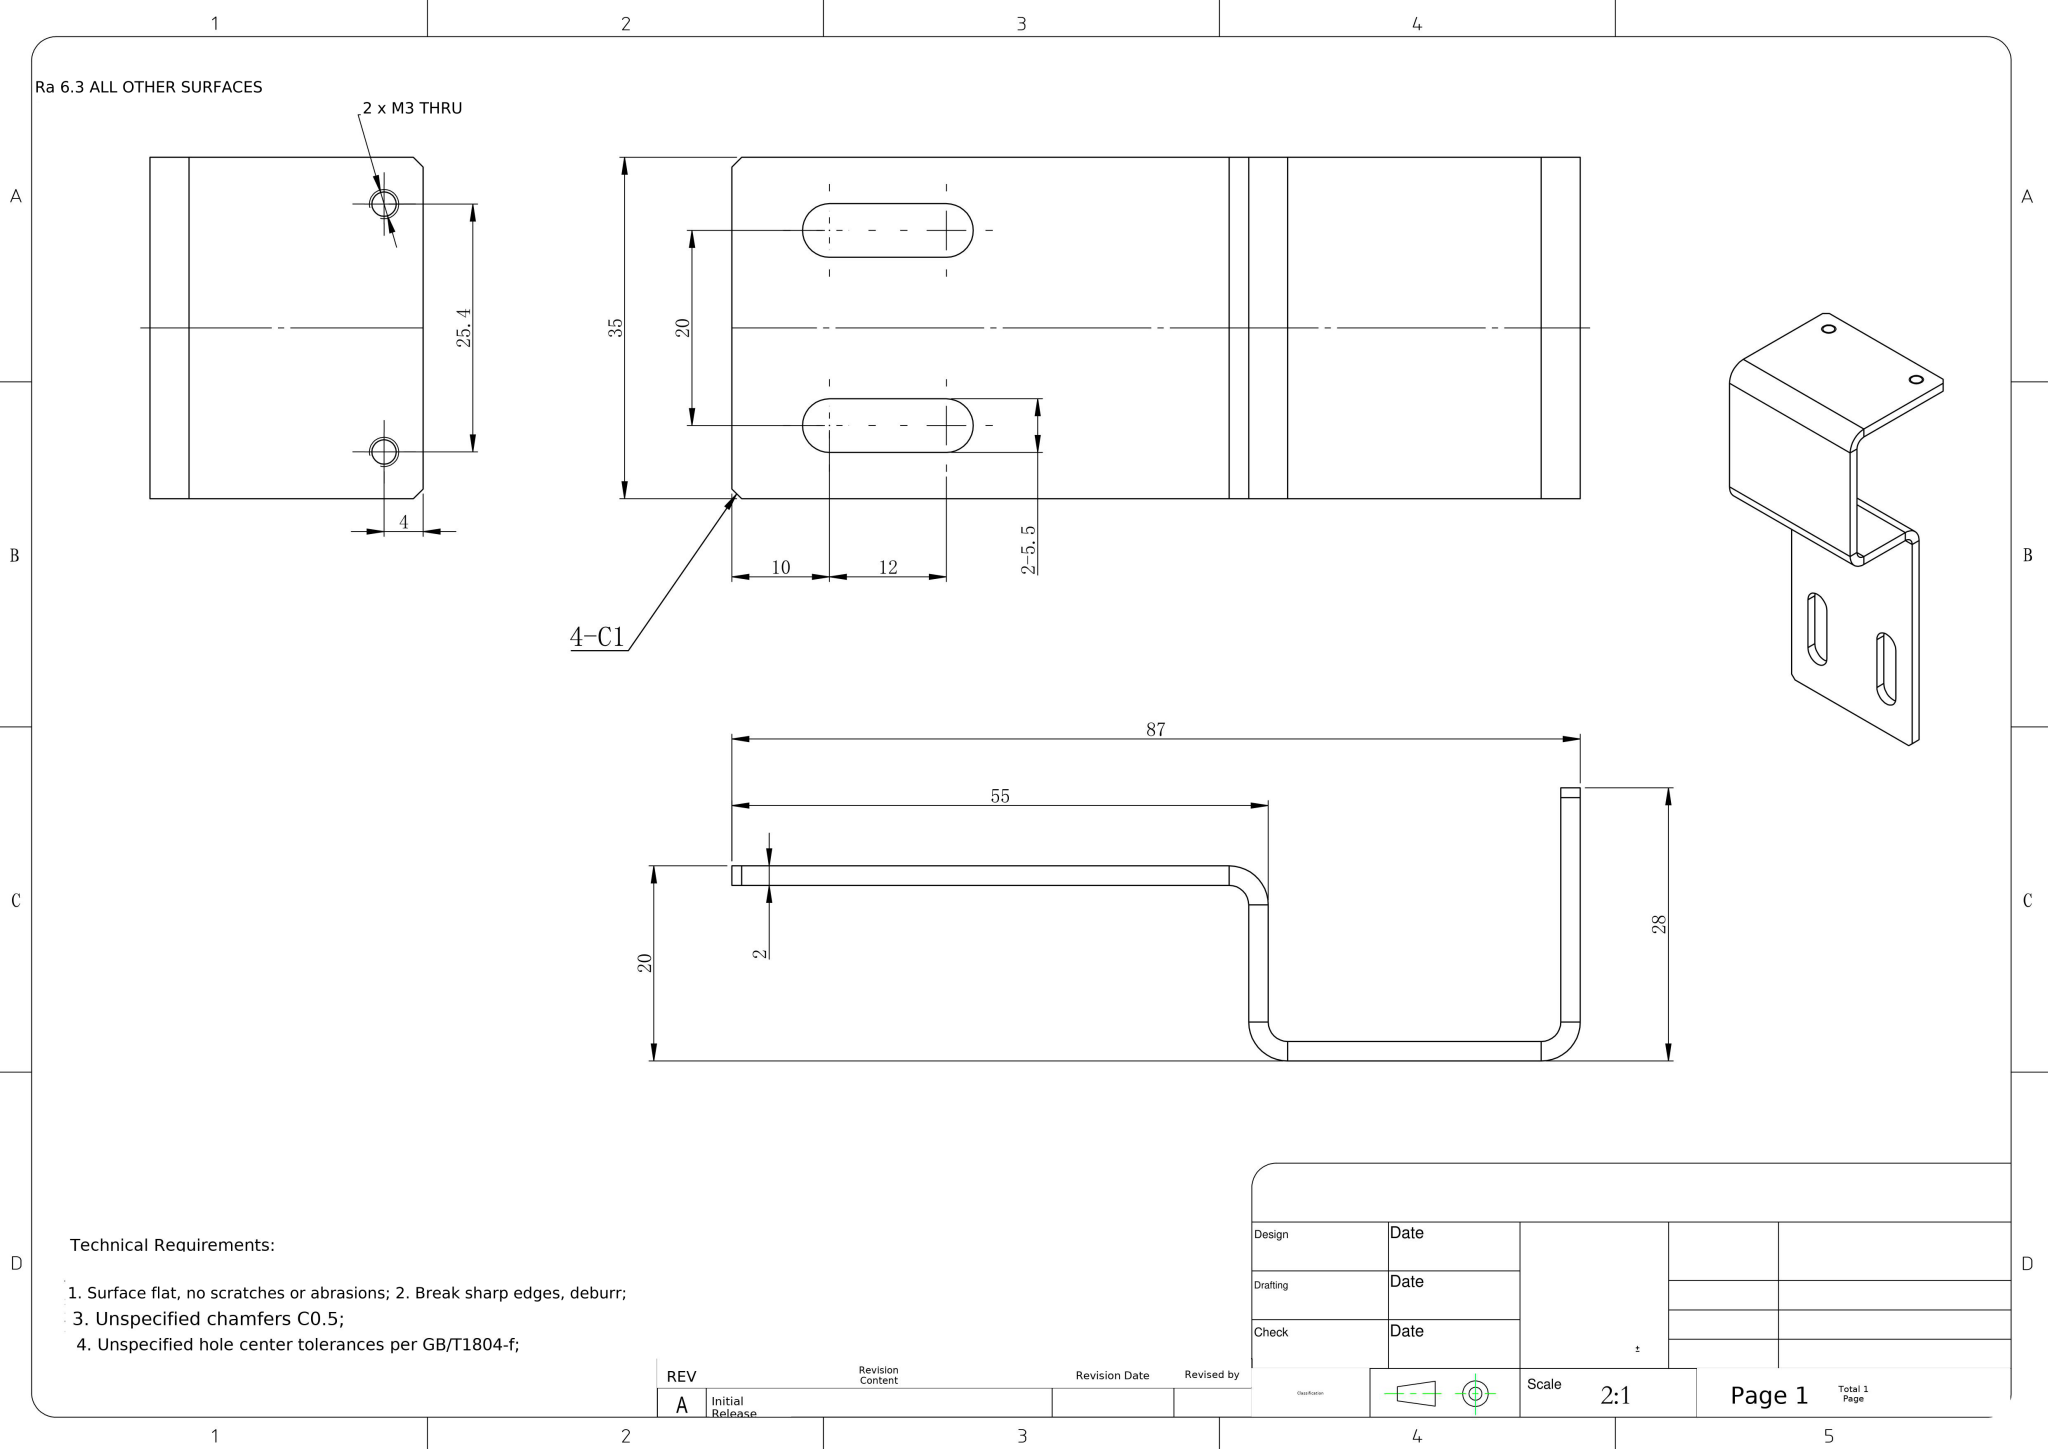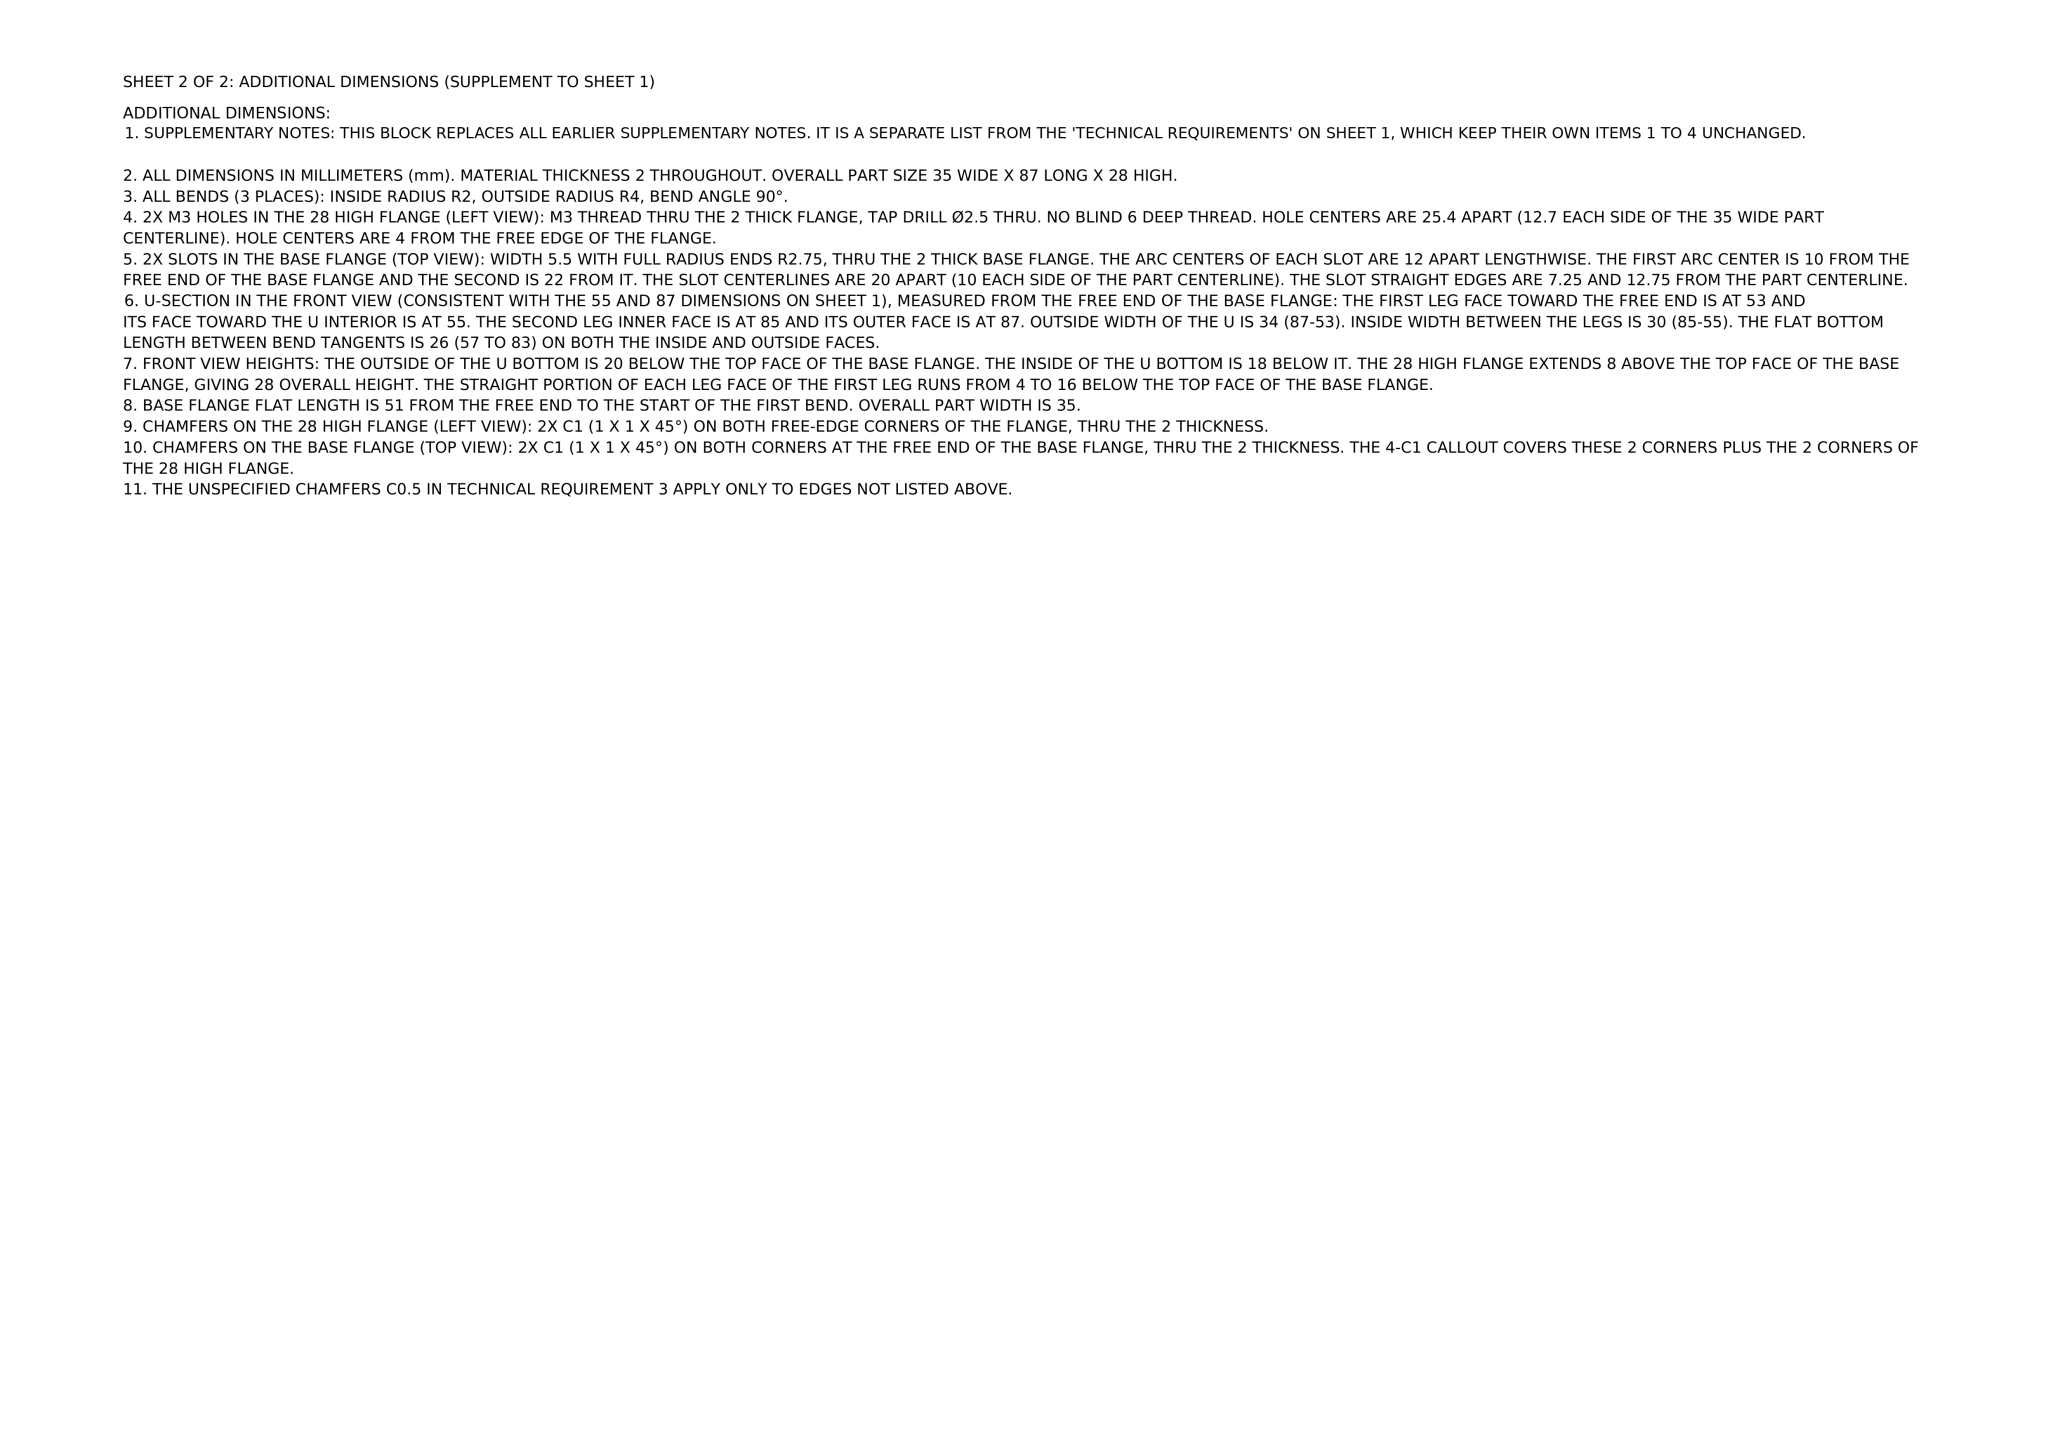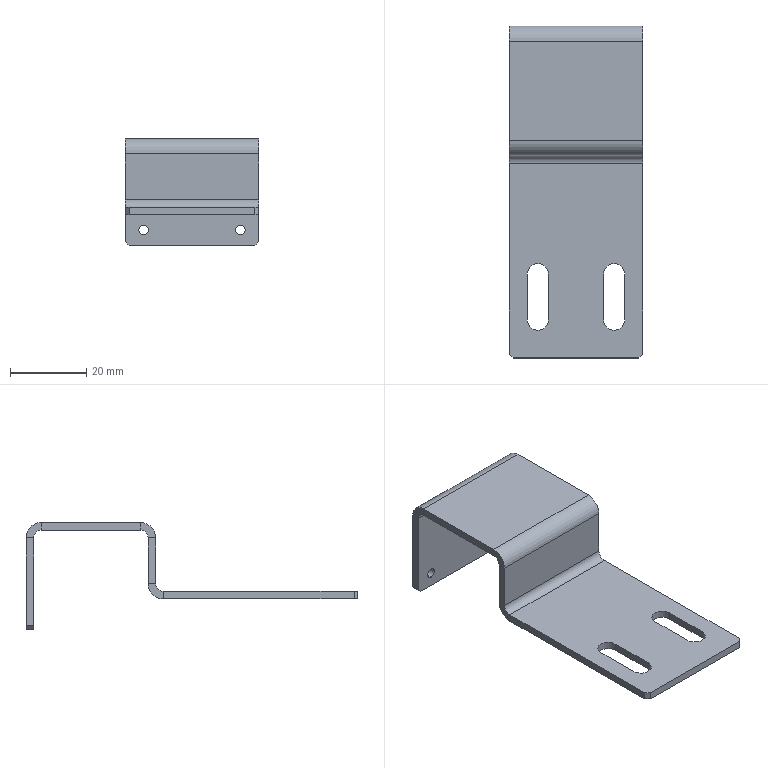Part | NX | mm | 1 solid | 46 faces | box 35 x 87 x 28 mm | volume 8517 mm3 | plane 32 | cylinder 14 | commonest cylinder face diameters 2.5 x4 5.5 x4 8 x3 4 x3